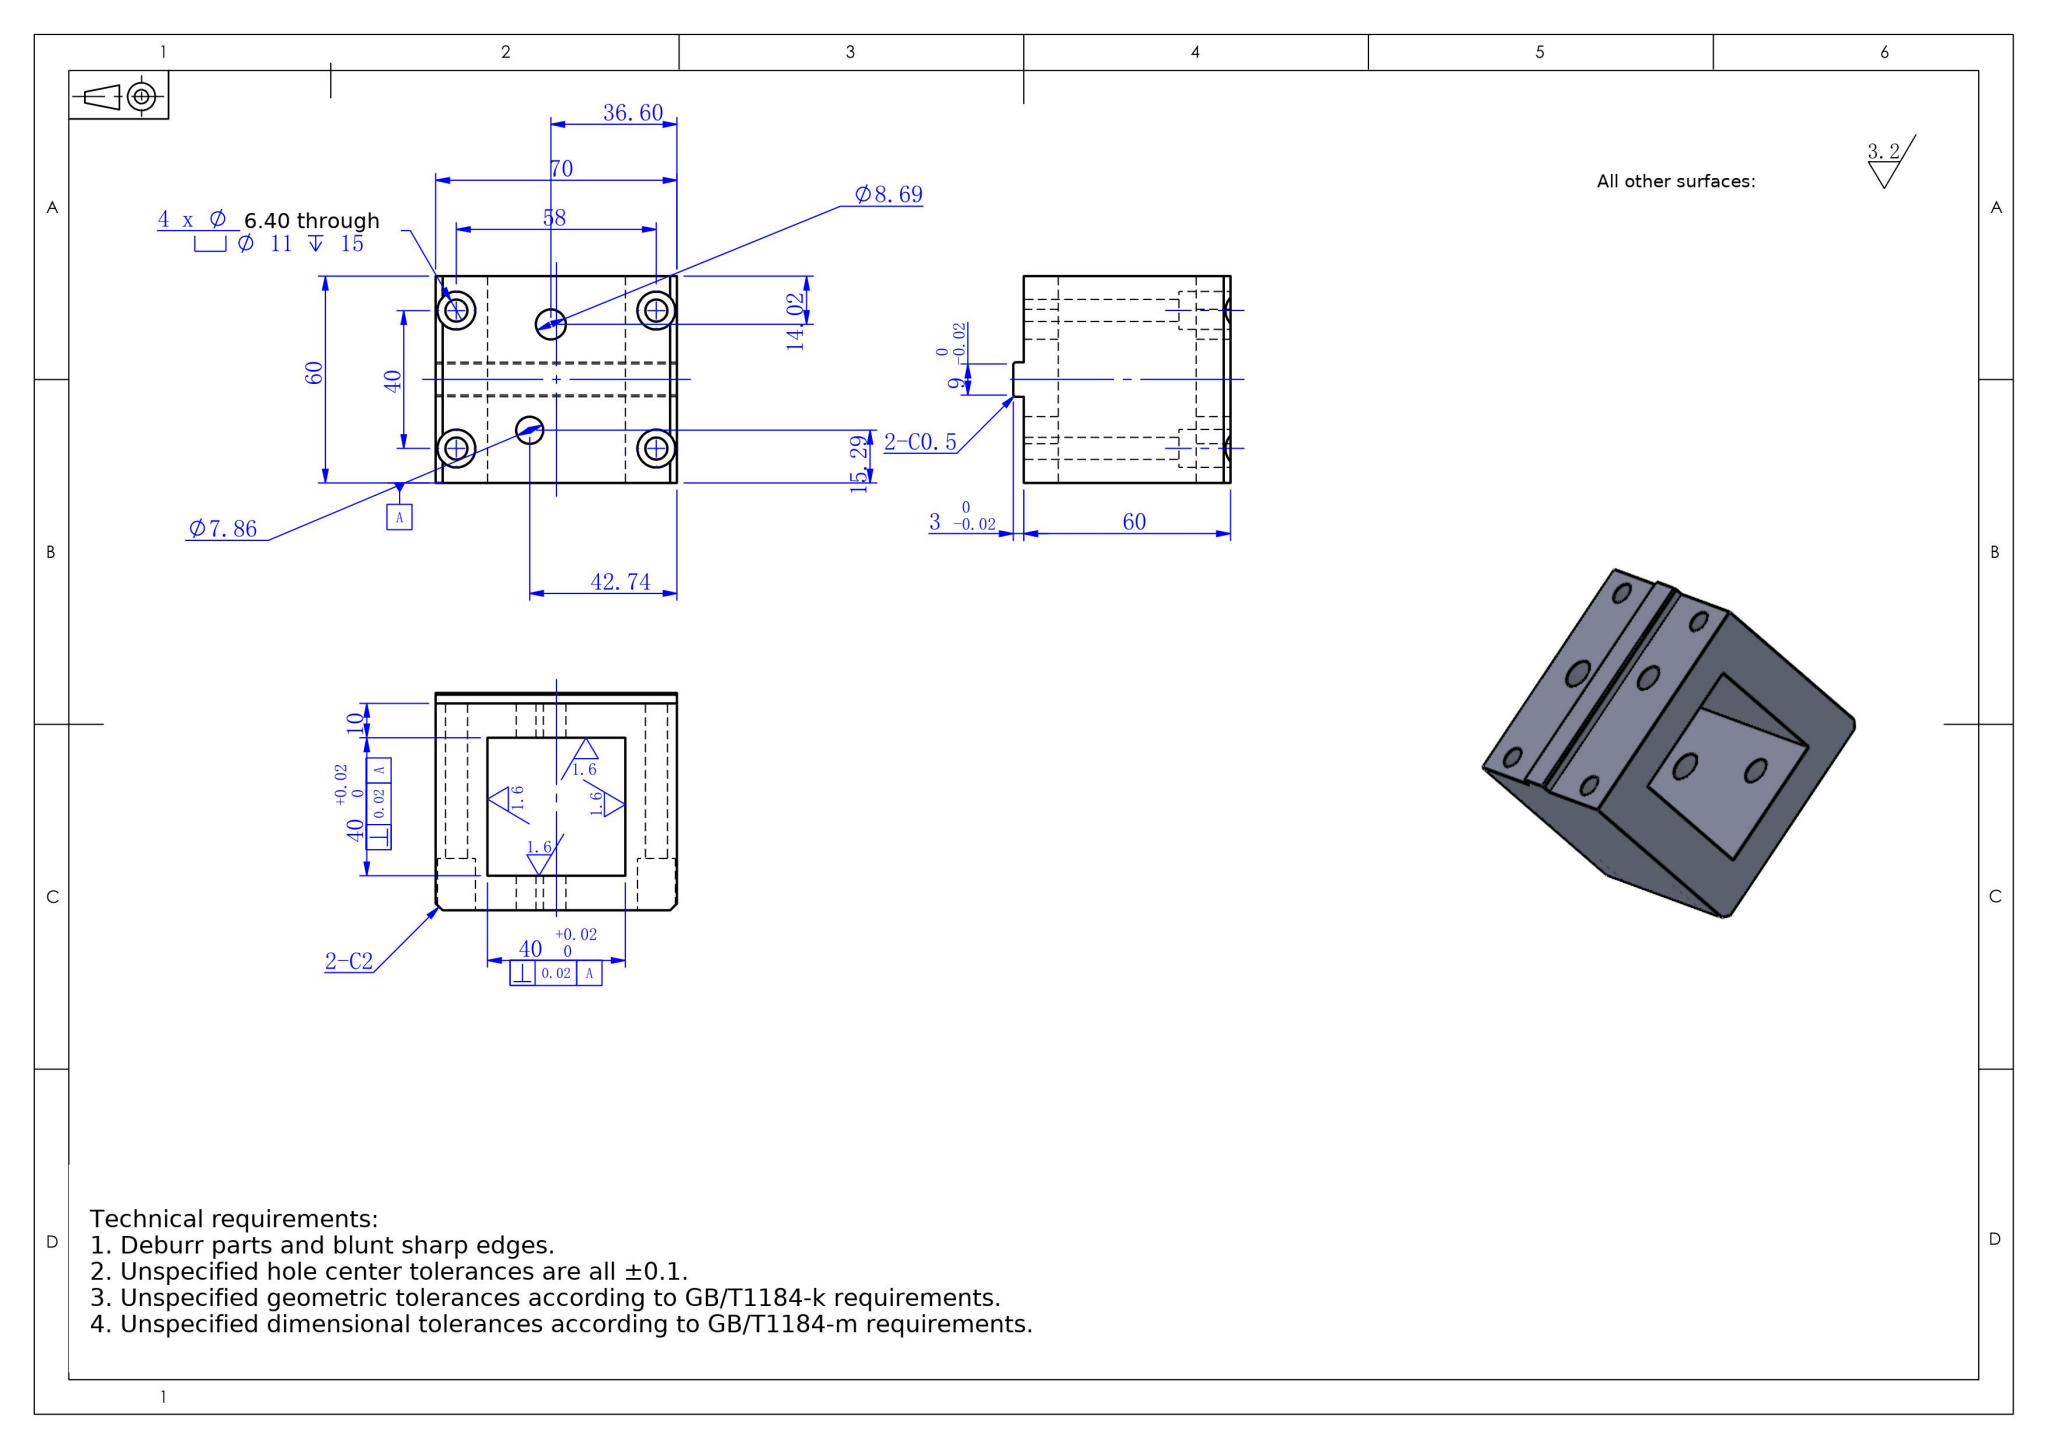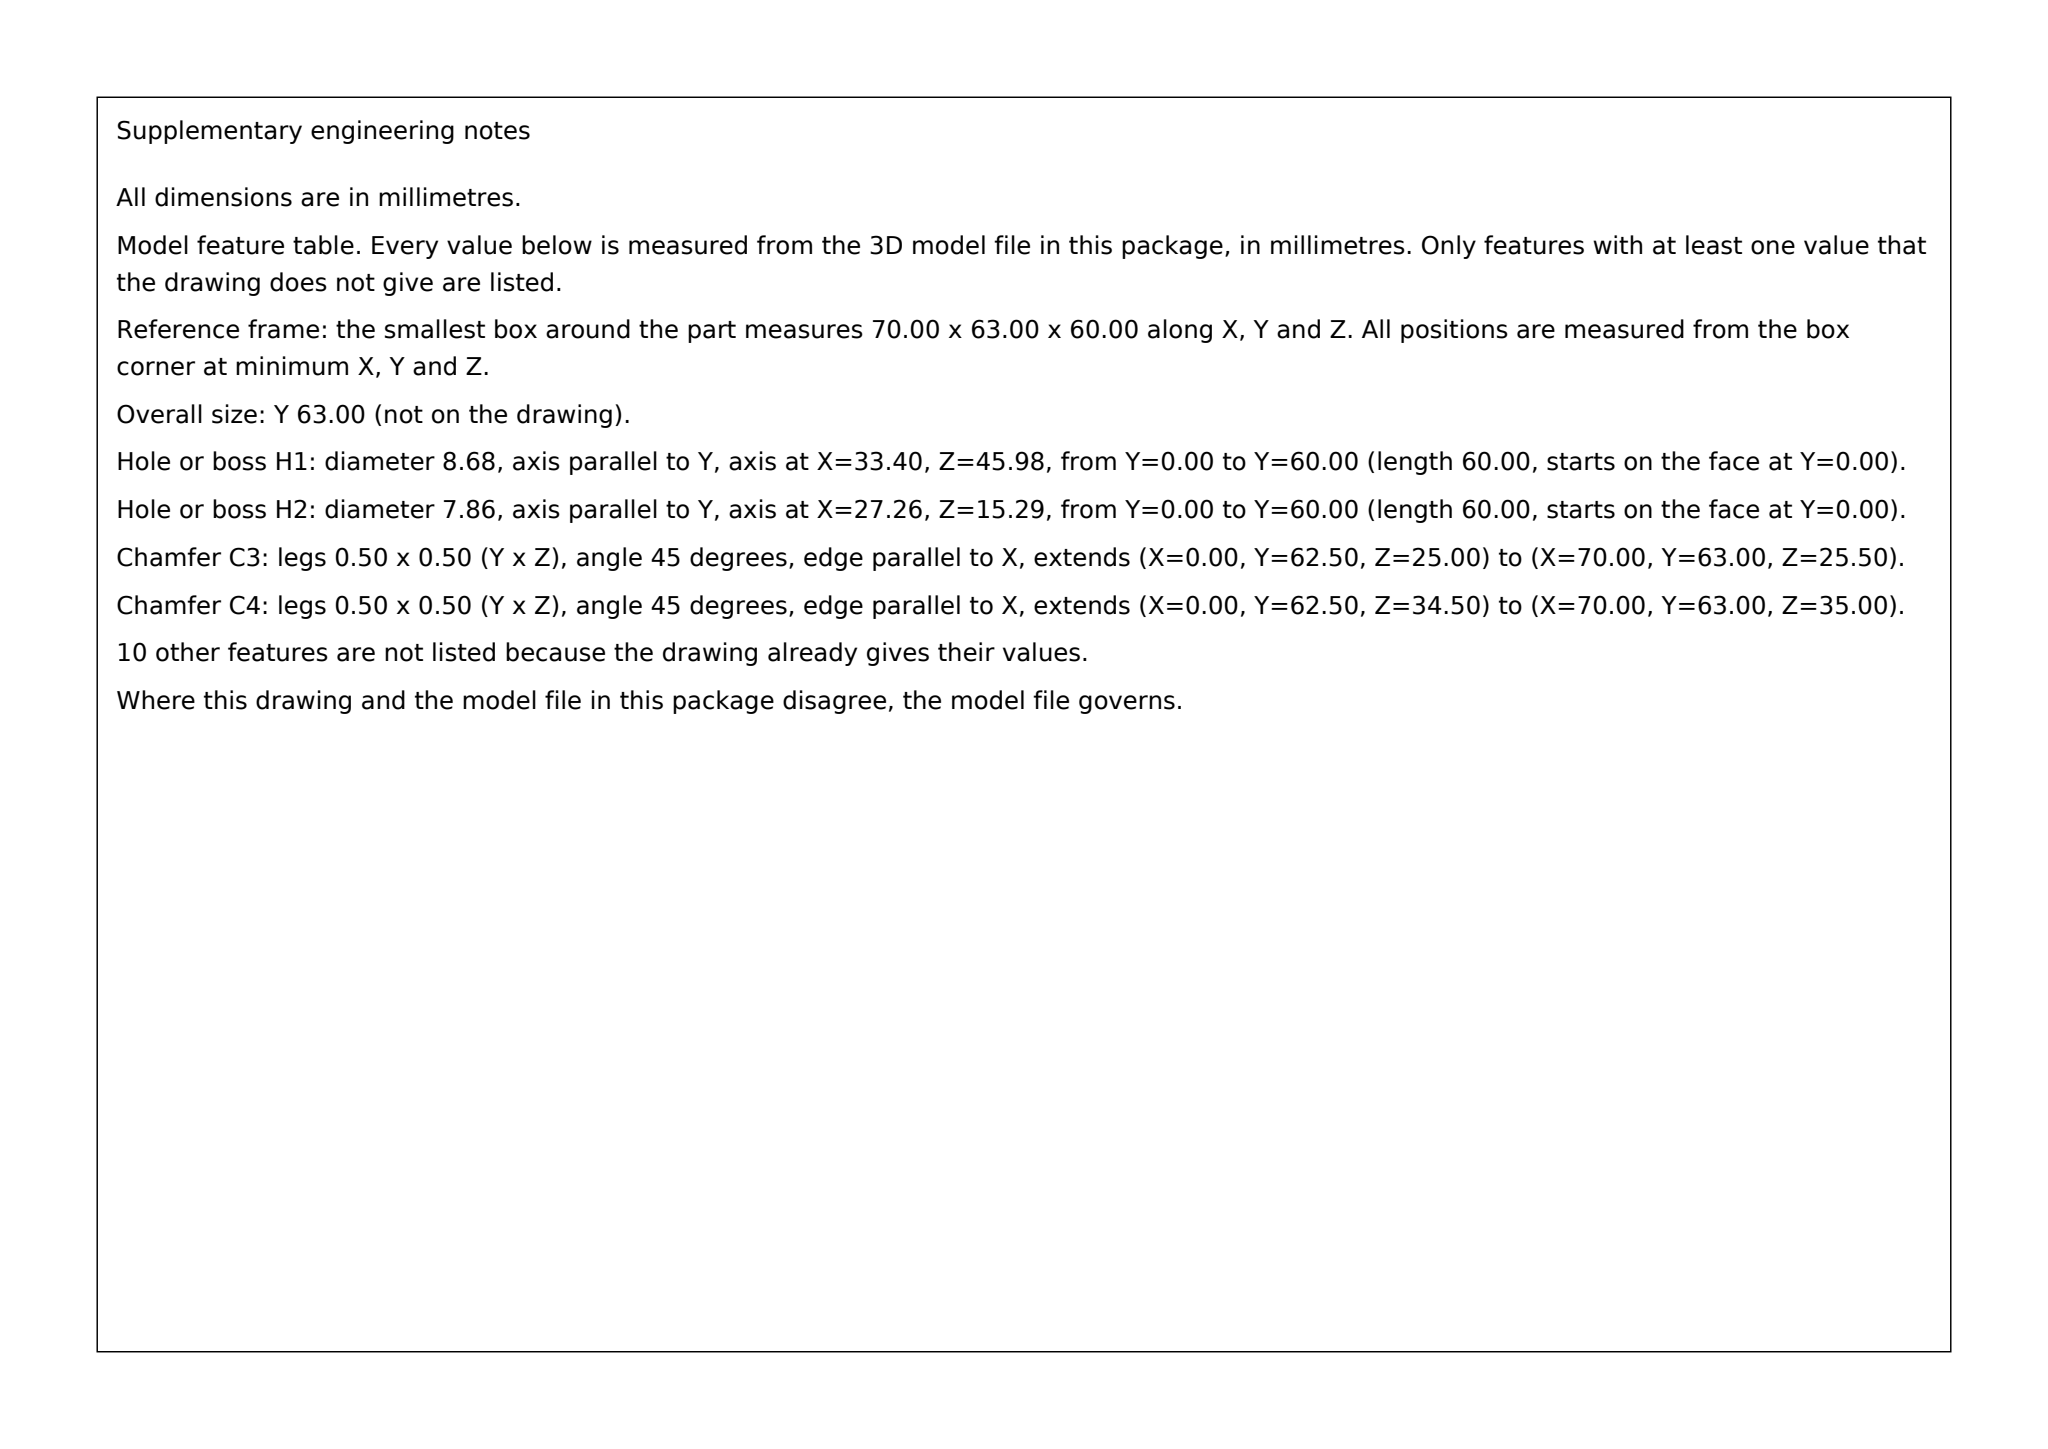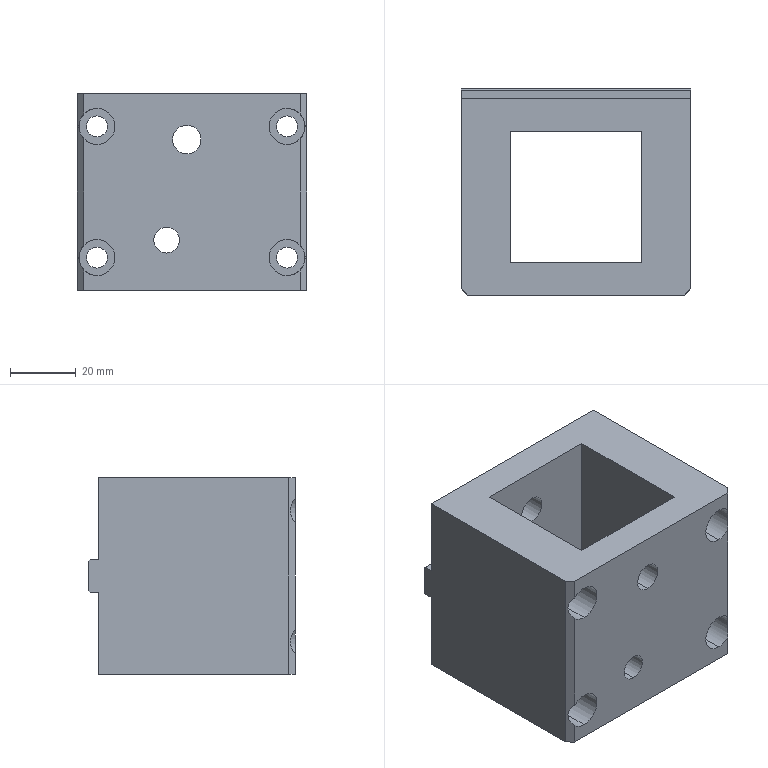Part | SolidWorks | mm | 1 solid | 46 faces | box 70 x 63 x 60 mm | volume 144212 mm3 | cylinder 24 | plane 22 | commonest cylinder face diameters 11 x8 6.4 x8 7.863 x4 8.688 x4